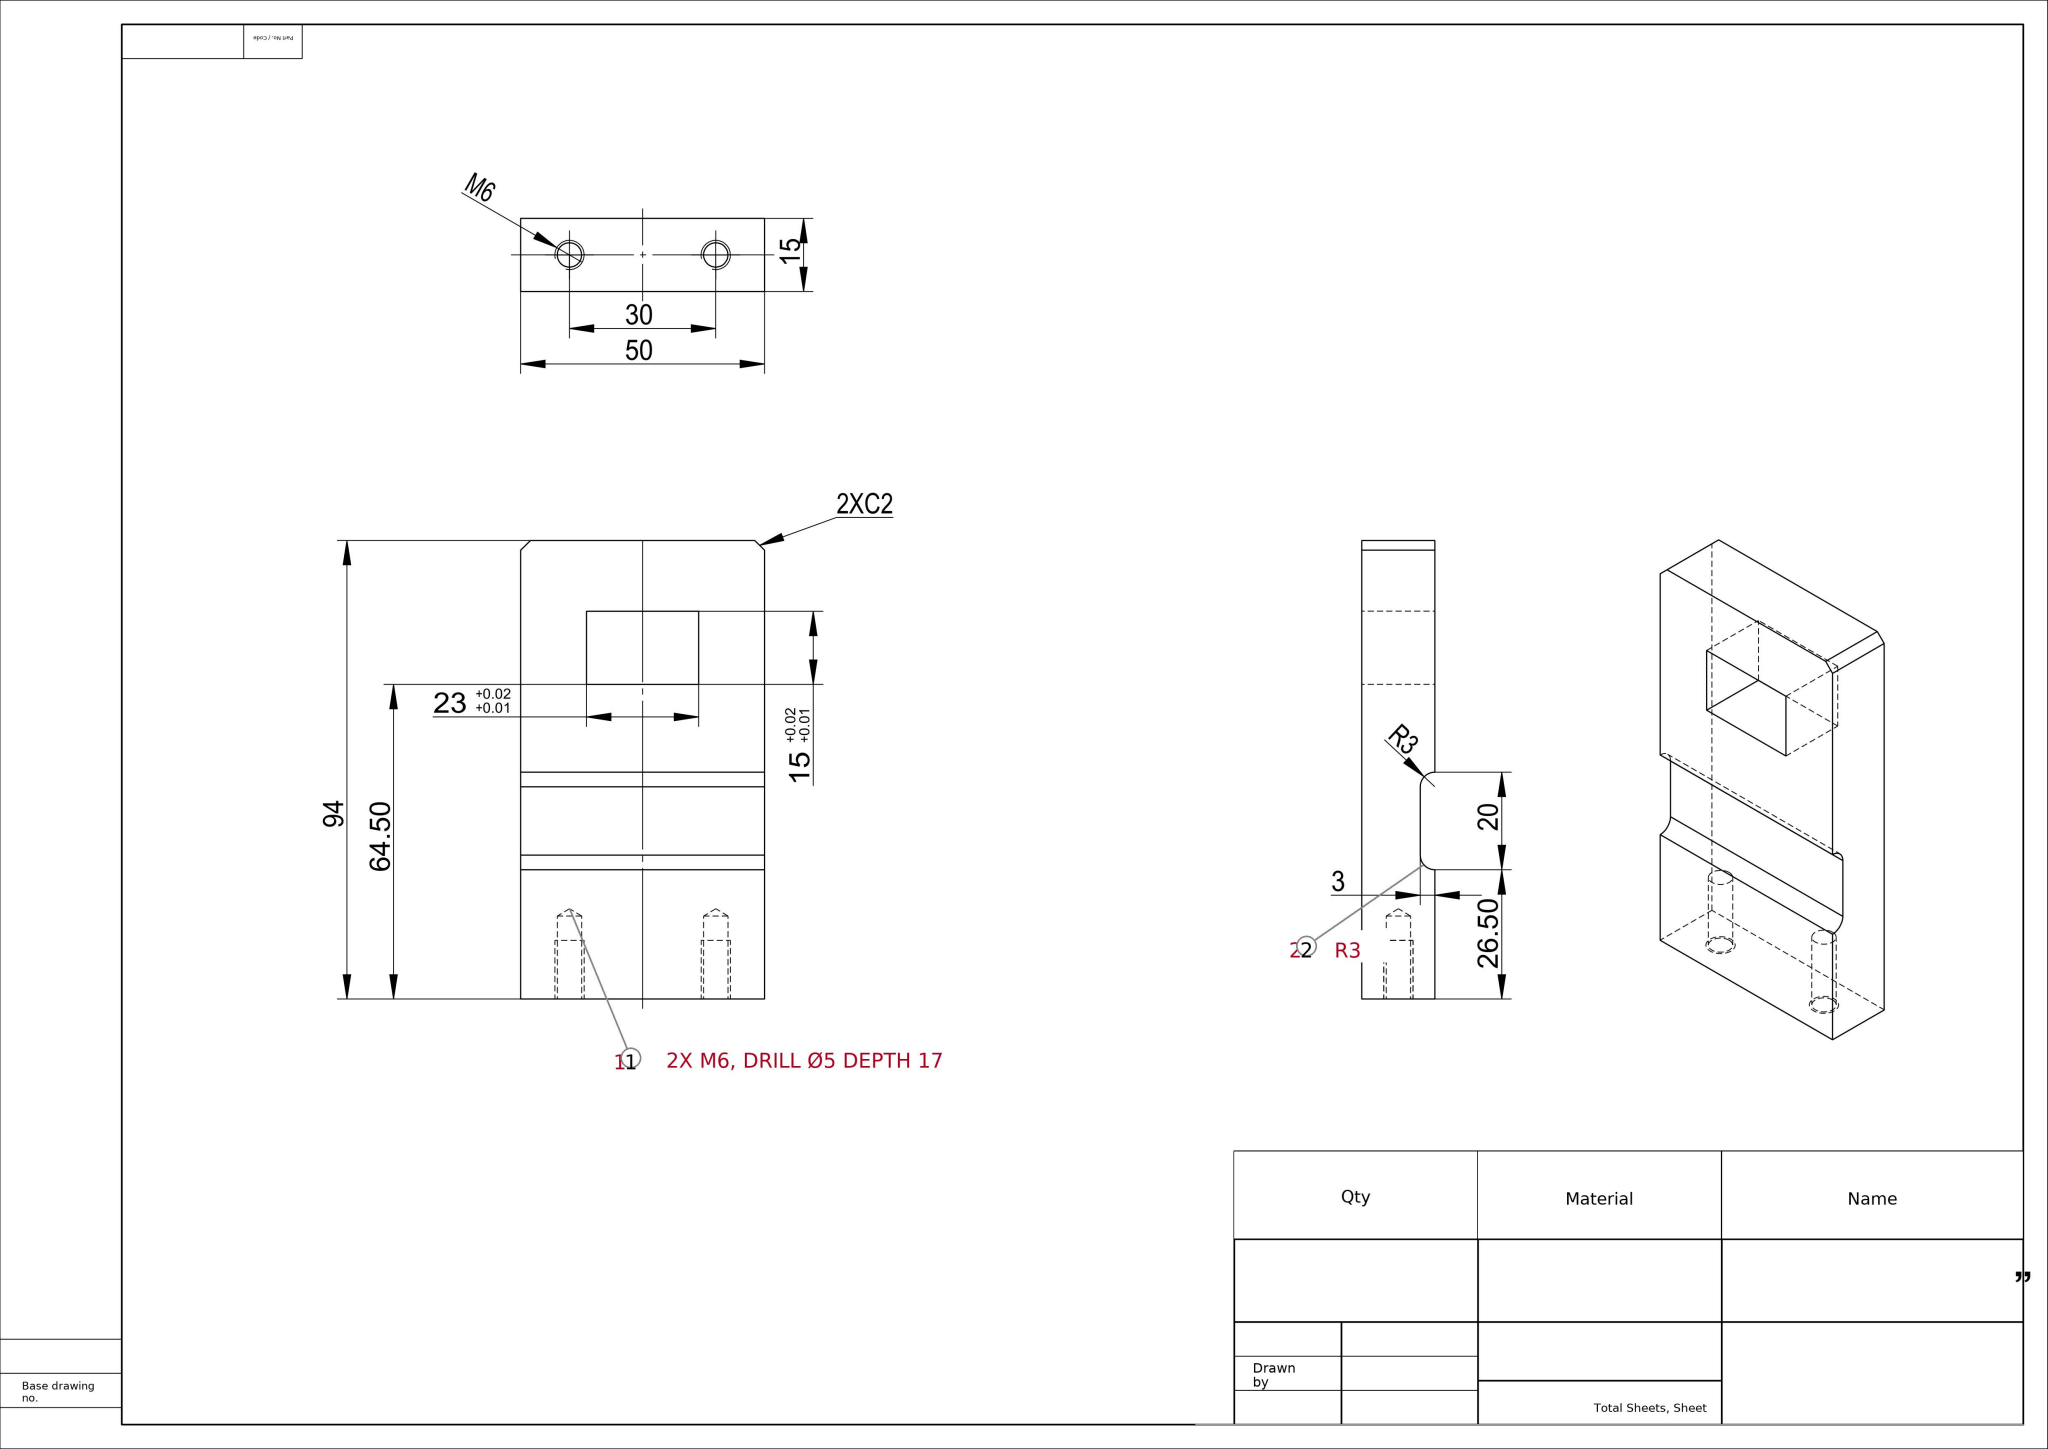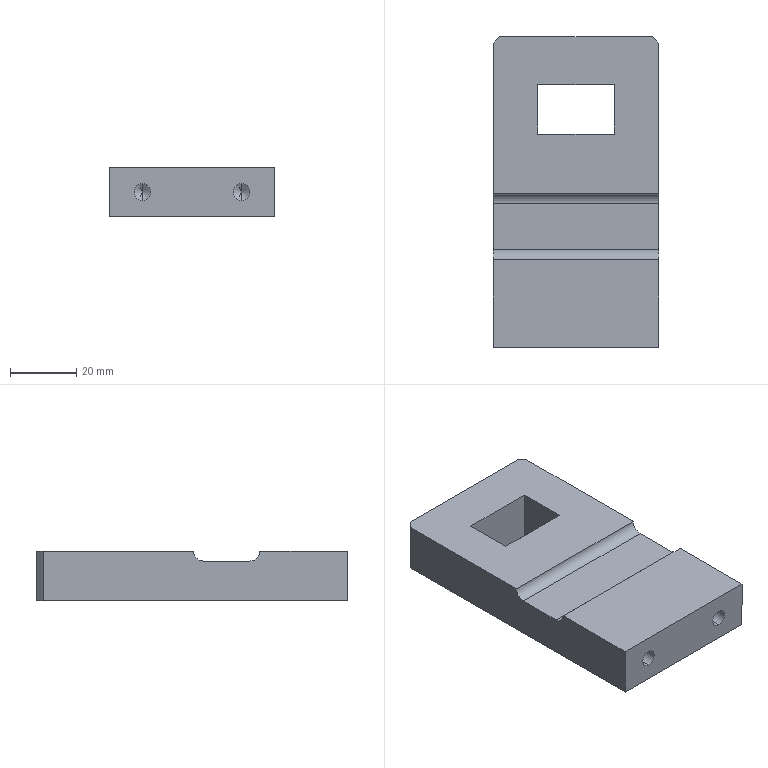Part | SolidWorks | mm | 1 solid | 24 faces | box 50 x 94 x 15 mm | volume 61771 mm3 | plane 14 | cylinder 6 | cone 4 | commonest cylinder face diameters 5 x4 6 x2
STEP:
#1=CARTESIAN_POINT('',(-15.,27.,2.5));
#2=VERTEX_POINT('',#1);
#3=CARTESIAN_POINT('',(-15.,27.,-2.5));
#4=VERTEX_POINT('',#3);
#5=CARTESIAN_POINT('',(-15.,27.,0.));
#6=DIRECTION('',(0.,-1.,0.));
#7=DIRECTION('',(0.,0.,-1.));
#8=AXIS2_PLACEMENT_3D('',#5,#6,#7);
#9=CIRCLE('',#8,2.5);
#10=EDGE_CURVE('',#2,#4,#9,.T.);
#11=ORIENTED_EDGE('',*,*,#10,.F.);
#12=CARTESIAN_POINT('',(-15.,10.,2.5));
#13=VERTEX_POINT('',#12);
#14=CARTESIAN_POINT('',(-15.,10.,2.5));
#15=DIRECTION('',(0.,-1.,0.));
#16=VECTOR('',#15,1000.);
#17=LINE('',#14,#16);
#18=EDGE_CURVE('',#2,#13,#17,.T.);
#19=ORIENTED_EDGE('',*,*,#18,.T.);
#20=CARTESIAN_POINT('',(-15.,10.,-2.5));
#21=VERTEX_POINT('',#20);
#22=CARTESIAN_POINT('',(-15.,10.,0.));
#23=DIRECTION('',(0.,-1.,0.));
#24=DIRECTION('',(0.,0.,-1.));
#25=AXIS2_PLACEMENT_3D('',#22,#23,#24);
#26=CIRCLE('',#25,2.5);
#27=EDGE_CURVE('',#13,#21,#26,.T.);
#28=ORIENTED_EDGE('',*,*,#27,.T.);
#29=CARTESIAN_POINT('',(-15.,10.,-2.5));
#30=DIRECTION('',(0.,-1.,0.));
#31=VECTOR('',#30,1000.);
#32=LINE('',#29,#31);
#33=EDGE_CURVE('',#4,#21,#32,.T.);
#34=ORIENTED_EDGE('',*,*,#33,.F.);
#35=EDGE_LOOP('',(#11,#19,#28,#34));
#36=FACE_OUTER_BOUND('',#35,.T.);
#37=CARTESIAN_POINT('',(-15.,10.,0.));
#38=DIRECTION('',(0.,-1.,0.));
#39=DIRECTION('',(0.,0.,-1.));
#40=AXIS2_PLACEMENT_3D('',#37,#38,#39);
#41=CYLINDRICAL_SURFACE('',#40,2.5);
#42=ADVANCED_FACE('',(#36),#41,.F.);
#43=CARTESIAN_POINT('',(-15.,28.502,0.));
#44=VERTEX_POINT('',#43);
#45=CARTESIAN_POINT('',(-15.,27.,-2.5));
#46=DIRECTION('',(0.,-0.515,-0.8572));
#47=VECTOR('',#46,1000.);
#48=LINE('',#45,#47);
#49=EDGE_CURVE('',#44,#4,#48,.T.);
#50=ORIENTED_EDGE('',*,*,#49,.F.);
#51=CARTESIAN_POINT('',(-15.,27.,2.5));
#52=DIRECTION('',(0.,-0.515,0.8572));
#53=VECTOR('',#52,1000.);
#54=LINE('',#51,#53);
#55=EDGE_CURVE('',#44,#2,#54,.T.);
#56=ORIENTED_EDGE('',*,*,#55,.T.);
#57=ORIENTED_EDGE('',*,*,#10,.T.);
#58=EDGE_LOOP('',(#50,#56,#57));
#59=FACE_OUTER_BOUND('',#58,.T.);
#60=CARTESIAN_POINT('',(-15.,27.,0.));
#61=DIRECTION('',(0.,-1.,0.));
#62=DIRECTION('',(0.,0.,-1.));
#63=AXIS2_PLACEMENT_3D('',#60,#61,#62);
#64=CONICAL_SURFACE('',#63,2.5,1.03);
#65=ADVANCED_FACE('',(#59),#64,.F.);
#66=CARTESIAN_POINT('',(15.,27.,2.5));
#67=VERTEX_POINT('',#66);
#68=CARTESIAN_POINT('',(15.,27.,-2.5));
#69=VERTEX_POINT('',#68);
#70=CARTESIAN_POINT('',(15.,27.,0.));
#71=DIRECTION('',(0.,-1.,0.));
#72=DIRECTION('',(0.,0.,-1.));
#73=AXIS2_PLACEMENT_3D('',#70,#71,#72);
#74=CIRCLE('',#73,2.5);
#75=EDGE_CURVE('',#67,#69,#74,.T.);
#76=ORIENTED_EDGE('',*,*,#75,.F.);
#77=CARTESIAN_POINT('',(15.,10.,2.5));
#78=VERTEX_POINT('',#77);
#79=CARTESIAN_POINT('',(15.,10.,2.5));
#80=DIRECTION('',(0.,-1.,0.));
#81=VECTOR('',#80,1000.);
#82=LINE('',#79,#81);
#83=EDGE_CURVE('',#67,#78,#82,.T.);
#84=ORIENTED_EDGE('',*,*,#83,.T.);
#85=CARTESIAN_POINT('',(15.,10.,-2.5));
#86=VERTEX_POINT('',#85);
#87=CARTESIAN_POINT('',(15.,10.,0.));
#88=DIRECTION('',(0.,-1.,0.));
#89=DIRECTION('',(0.,0.,-1.));
#90=AXIS2_PLACEMENT_3D('',#87,#88,#89);
#91=CIRCLE('',#90,2.5);
#92=EDGE_CURVE('',#78,#86,#91,.T.);
#93=ORIENTED_EDGE('',*,*,#92,.T.);
#94=CARTESIAN_POINT('',(15.,10.,-2.5));
#95=DIRECTION('',(0.,-1.,0.));
#96=VECTOR('',#95,1000.);
#97=LINE('',#94,#96);
#98=EDGE_CURVE('',#69,#86,#97,.T.);
#99=ORIENTED_EDGE('',*,*,#98,.F.);
#100=EDGE_LOOP('',(#76,#84,#93,#99));
#101=FACE_OUTER_BOUND('',#100,.T.);
#102=CARTESIAN_POINT('',(15.,10.,0.));
#103=DIRECTION('',(0.,-1.,0.));
#104=DIRECTION('',(0.,0.,-1.));
#105=AXIS2_PLACEMENT_3D('',#102,#103,#104);
#106=CYLINDRICAL_SURFACE('',#105,2.5);
#107=ADVANCED_FACE('',(#101),#106,.F.);
#108=CARTESIAN_POINT('',(15.,28.502,0.));
#109=VERTEX_POINT('',#108);
#110=CARTESIAN_POINT('',(15.,27.,-2.5));
#111=DIRECTION('',(0.,-0.515,-0.8572));
#112=VECTOR('',#111,1000.);
#113=LINE('',#110,#112);
#114=EDGE_CURVE('',#109,#69,#113,.T.);
#115=ORIENTED_EDGE('',*,*,#114,.F.);
#116=CARTESIAN_POINT('',(15.,27.,2.5));
#117=DIRECTION('',(0.,-0.515,0.8572));
#118=VECTOR('',#117,1000.);
#119=LINE('',#116,#118);
#120=EDGE_CURVE('',#109,#67,#119,.T.);
#121=ORIENTED_EDGE('',*,*,#120,.T.);
#122=ORIENTED_EDGE('',*,*,#75,.T.);
#123=EDGE_LOOP('',(#115,#121,#122));
#124=FACE_OUTER_BOUND('',#123,.T.);
#125=CARTESIAN_POINT('',(15.,27.,0.));
#126=DIRECTION('',(0.,-1.,0.));
#127=DIRECTION('',(0.,0.,-1.));
#128=AXIS2_PLACEMENT_3D('',#125,#126,#127);
#129=CONICAL_SURFACE('',#128,2.5,1.03);
#130=ADVANCED_FACE('',(#124),#129,.F.);
#131=CARTESIAN_POINT('',(25.,102.,-7.5));
#132=VERTEX_POINT('',#131);
#133=CARTESIAN_POINT('',(25.,10.,-7.5));
#134=VERTEX_POINT('',#133);
#135=CARTESIAN_POINT('',(25.,120.,-7.5));
#136=DIRECTION('',(0.,-1.,0.));
#137=VECTOR('',#136,1000.);
#138=LINE('',#135,#137);
#139=EDGE_CURVE('',#132,#134,#138,.T.);
#140=ORIENTED_EDGE('',*,*,#139,.F.);
#141=CARTESIAN_POINT('',(25.,102.,7.5));
#142=VERTEX_POINT('',#141);
#143=CARTESIAN_POINT('',(25.,102.,-7.5));
#144=DIRECTION('',(0.,0.,1.));
#145=VECTOR('',#144,1000.);
#146=LINE('',#143,#145);
#147=EDGE_CURVE('',#132,#142,#146,.T.);
#148=ORIENTED_EDGE('',*,*,#147,.T.);
#149=CARTESIAN_POINT('',(25.,56.5,7.5));
#150=VERTEX_POINT('',#149);
#151=CARTESIAN_POINT('',(25.,120.,7.5));
#152=DIRECTION('',(0.,-1.,0.));
#153=VECTOR('',#152,1000.);
#154=LINE('',#151,#153);
#155=EDGE_CURVE('',#142,#150,#154,.T.);
#156=ORIENTED_EDGE('',*,*,#155,.T.);
#157=CARTESIAN_POINT('',(25.,53.5,4.5));
#158=VERTEX_POINT('',#157);
#159=CARTESIAN_POINT('',(25.,53.5,7.5));
#160=DIRECTION('',(-1.,0.,0.));
#161=DIRECTION('',(0.,0.,1.));
#162=AXIS2_PLACEMENT_3D('',#159,#160,#161);
#163=CIRCLE('',#162,3.);
#164=EDGE_CURVE('',#150,#158,#163,.T.);
#165=ORIENTED_EDGE('',*,*,#164,.T.);
#166=CARTESIAN_POINT('',(25.,39.5,4.5));
#167=VERTEX_POINT('',#166);
#168=CARTESIAN_POINT('',(25.,56.5,4.5));
#169=DIRECTION('',(-0.,-1.,0.));
#170=VECTOR('',#169,1000.);
#171=LINE('',#168,#170);
#172=EDGE_CURVE('',#158,#167,#171,.T.);
#173=ORIENTED_EDGE('',*,*,#172,.T.);
#174=CARTESIAN_POINT('',(25.,36.5,7.5));
#175=VERTEX_POINT('',#174);
#176=CARTESIAN_POINT('',(25.,39.5,7.5));
#177=DIRECTION('',(-1.,0.,0.));
#178=DIRECTION('',(0.,0.,1.));
#179=AXIS2_PLACEMENT_3D('',#176,#177,#178);
#180=CIRCLE('',#179,3.);
#181=EDGE_CURVE('',#167,#175,#180,.T.);
#182=ORIENTED_EDGE('',*,*,#181,.T.);
#183=CARTESIAN_POINT('',(25.,10.,7.5));
#184=VERTEX_POINT('',#183);
#185=CARTESIAN_POINT('',(25.,120.,7.5));
#186=DIRECTION('',(0.,-1.,0.));
#187=VECTOR('',#186,1000.);
#188=LINE('',#185,#187);
#189=EDGE_CURVE('',#175,#184,#188,.T.);
#190=ORIENTED_EDGE('',*,*,#189,.T.);
#191=CARTESIAN_POINT('',(25.,10.,7.5));
#192=DIRECTION('',(0.,0.,-1.));
#193=VECTOR('',#192,1000.);
#194=LINE('',#191,#193);
#195=EDGE_CURVE('',#184,#134,#194,.T.);
#196=ORIENTED_EDGE('',*,*,#195,.T.);
#197=EDGE_LOOP('',(#140,#148,#156,#165,#173,#182,#190,#196));
#198=FACE_OUTER_BOUND('',#197,.T.);
#199=CARTESIAN_POINT('',(25.,120.,-7.5));
#200=DIRECTION('',(-1.,0.,0.));
#201=DIRECTION('',(0.,0.,1.));
#202=AXIS2_PLACEMENT_3D('',#199,#200,#201);
#203=PLANE('',#202);
#204=ADVANCED_FACE('',(#198),#203,.F.);
#205=CARTESIAN_POINT('',(-25.,102.,7.5));
#206=VERTEX_POINT('',#205);
#207=CARTESIAN_POINT('',(-25.,56.5,7.5));
#208=VERTEX_POINT('',#207);
#209=CARTESIAN_POINT('',(-25.,120.,7.5));
#210=DIRECTION('',(0.,-1.,0.));
#211=VECTOR('',#210,1000.);
#212=LINE('',#209,#211);
#213=EDGE_CURVE('',#206,#208,#212,.T.);
#214=ORIENTED_EDGE('',*,*,#213,.F.);
#215=CARTESIAN_POINT('',(-25.,102.,-7.5));
#216=VERTEX_POINT('',#215);
#217=CARTESIAN_POINT('',(-25.,102.,-7.5));
#218=DIRECTION('',(0.,0.,-1.));
#219=VECTOR('',#218,1000.);
#220=LINE('',#217,#219);
#221=EDGE_CURVE('',#206,#216,#220,.T.);
#222=ORIENTED_EDGE('',*,*,#221,.T.);
#223=CARTESIAN_POINT('',(-25.,10.,-7.5));
#224=VERTEX_POINT('',#223);
#225=CARTESIAN_POINT('',(-25.,120.,-7.5));
#226=DIRECTION('',(0.,-1.,0.));
#227=VECTOR('',#226,1000.);
#228=LINE('',#225,#227);
#229=EDGE_CURVE('',#216,#224,#228,.T.);
#230=ORIENTED_EDGE('',*,*,#229,.T.);
#231=CARTESIAN_POINT('',(-25.,10.,7.5));
#232=VERTEX_POINT('',#231);
#233=CARTESIAN_POINT('',(-25.,10.,7.5));
#234=DIRECTION('',(0.,0.,-1.));
#235=VECTOR('',#234,1000.);
#236=LINE('',#233,#235);
#237=EDGE_CURVE('',#232,#224,#236,.T.);
#238=ORIENTED_EDGE('',*,*,#237,.F.);
#239=CARTESIAN_POINT('',(-25.,36.5,7.5));
#240=VERTEX_POINT('',#239);
#241=CARTESIAN_POINT('',(-25.,120.,7.5));
#242=DIRECTION('',(0.,-1.,0.));
#243=VECTOR('',#242,1000.);
#244=LINE('',#241,#243);
#245=EDGE_CURVE('',#240,#232,#244,.T.);
#246=ORIENTED_EDGE('',*,*,#245,.F.);
#247=CARTESIAN_POINT('',(-25.,39.5,4.5));
#248=VERTEX_POINT('',#247);
#249=CARTESIAN_POINT('',(-25.,39.5,7.5));
#250=DIRECTION('',(1.,0.,0.));
#251=DIRECTION('',(0.,0.,-1.));
#252=AXIS2_PLACEMENT_3D('',#249,#250,#251);
#253=CIRCLE('',#252,3.);
#254=EDGE_CURVE('',#240,#248,#253,.T.);
#255=ORIENTED_EDGE('',*,*,#254,.T.);
#256=CARTESIAN_POINT('',(-25.,53.5,4.5));
#257=VERTEX_POINT('',#256);
#258=CARTESIAN_POINT('',(-25.,56.5,4.5));
#259=DIRECTION('',(0.,1.,0.));
#260=VECTOR('',#259,1000.);
#261=LINE('',#258,#260);
#262=EDGE_CURVE('',#248,#257,#261,.T.);
#263=ORIENTED_EDGE('',*,*,#262,.T.);
#264=CARTESIAN_POINT('',(-25.,53.5,7.5));
#265=DIRECTION('',(1.,0.,0.));
#266=DIRECTION('',(0.,0.,-1.));
#267=AXIS2_PLACEMENT_3D('',#264,#265,#266);
#268=CIRCLE('',#267,3.);
#269=EDGE_CURVE('',#257,#208,#268,.T.);
#270=ORIENTED_EDGE('',*,*,#269,.T.);
#271=EDGE_LOOP('',(#214,#222,#230,#238,#246,#255,#263,#270));
#272=FACE_OUTER_BOUND('',#271,.T.);
#273=CARTESIAN_POINT('',(-25.,120.,-7.5));
#274=DIRECTION('',(1.,0.,0.));
#275=DIRECTION('',(0.,0.,-1.));
#276=AXIS2_PLACEMENT_3D('',#273,#274,#275);
#277=PLANE('',#276);
#278=ADVANCED_FACE('',(#272),#277,.F.);
#279=CARTESIAN_POINT('',(25.,36.5,7.5));
#280=DIRECTION('',(-1.,0.,0.));
#281=VECTOR('',#280,1000.);
#282=LINE('',#279,#281);
#283=EDGE_CURVE('',#175,#240,#282,.T.);
#284=ORIENTED_EDGE('',*,*,#283,.T.);
#285=ORIENTED_EDGE('',*,*,#245,.T.);
#286=CARTESIAN_POINT('',(25.,10.,7.5));
#287=DIRECTION('',(1.,0.,0.));
#288=VECTOR('',#287,1000.);
#289=LINE('',#286,#288);
#290=EDGE_CURVE('',#232,#184,#289,.T.);
#291=ORIENTED_EDGE('',*,*,#290,.T.);
#292=ORIENTED_EDGE('',*,*,#189,.F.);
#293=EDGE_LOOP('',(#284,#285,#291,#292));
#294=FACE_OUTER_BOUND('',#293,.T.);
#295=CARTESIAN_POINT('',(-25.,120.,7.5));
#296=DIRECTION('',(0.,0.,-1.));
#297=DIRECTION('',(-1.,0.,0.));
#298=AXIS2_PLACEMENT_3D('',#295,#296,#297);
#299=PLANE('',#298);
#300=ADVANCED_FACE('',(#294),#299,.F.);
#301=CARTESIAN_POINT('',(-11.5,74.5,7.5));
#302=VERTEX_POINT('',#301);
#303=CARTESIAN_POINT('',(11.5,74.5,7.5));
#304=VERTEX_POINT('',#303);
#305=CARTESIAN_POINT('',(-11.5,74.5,7.5));
#306=DIRECTION('',(1.,0.,0.));
#307=VECTOR('',#306,1000.);
#308=LINE('',#305,#307);
#309=EDGE_CURVE('',#302,#304,#308,.T.);
#310=ORIENTED_EDGE('',*,*,#309,.F.);
#311=CARTESIAN_POINT('',(-11.5,89.5,7.5));
#312=VERTEX_POINT('',#311);
#313=CARTESIAN_POINT('',(-11.5,89.5,7.5));
#314=DIRECTION('',(0.,-1.,0.));
#315=VECTOR('',#314,1000.);
#316=LINE('',#313,#315);
#317=EDGE_CURVE('',#312,#302,#316,.T.);
#318=ORIENTED_EDGE('',*,*,#317,.F.);
#319=CARTESIAN_POINT('',(11.5,89.5,7.5));
#320=VERTEX_POINT('',#319);
#321=CARTESIAN_POINT('',(-11.5,89.5,7.5));
#322=DIRECTION('',(-1.,0.,0.));
#323=VECTOR('',#322,1000.);
#324=LINE('',#321,#323);
#325=EDGE_CURVE('',#320,#312,#324,.T.);
#326=ORIENTED_EDGE('',*,*,#325,.F.);
#327=CARTESIAN_POINT('',(11.5,89.5,7.5));
#328=DIRECTION('',(-0.,1.,0.));
#329=VECTOR('',#328,1000.);
#330=LINE('',#327,#329);
#331=EDGE_CURVE('',#304,#320,#330,.T.);
#332=ORIENTED_EDGE('',*,*,#331,.F.);
#333=EDGE_LOOP('',(#310,#318,#326,#332));
#334=FACE_BOUND('',#333,.T.);
#335=CARTESIAN_POINT('',(-23.,104.,7.5));
#336=VERTEX_POINT('',#335);
#337=CARTESIAN_POINT('',(23.,104.,7.5));
#338=VERTEX_POINT('',#337);
#339=CARTESIAN_POINT('',(-25.,104.,7.5));
#340=DIRECTION('',(1.,0.,0.));
#341=VECTOR('',#340,1000.);
#342=LINE('',#339,#341);
#343=EDGE_CURVE('',#336,#338,#342,.T.);
#344=ORIENTED_EDGE('',*,*,#343,.F.);
#345=CARTESIAN_POINT('',(-23.,104.,7.5));
#346=DIRECTION('',(-0.7071,-0.7071,0.));
#347=VECTOR('',#346,1000.);
#348=LINE('',#345,#347);
#349=EDGE_CURVE('',#336,#206,#348,.T.);
#350=ORIENTED_EDGE('',*,*,#349,.T.);
#351=ORIENTED_EDGE('',*,*,#213,.T.);
#352=CARTESIAN_POINT('',(25.,56.5,7.5));
#353=DIRECTION('',(1.,0.,0.));
#354=VECTOR('',#353,1000.);
#355=LINE('',#352,#354);
#356=EDGE_CURVE('',#208,#150,#355,.T.);
#357=ORIENTED_EDGE('',*,*,#356,.T.);
#358=ORIENTED_EDGE('',*,*,#155,.F.);
#359=CARTESIAN_POINT('',(25.,102.,7.5));
#360=DIRECTION('',(-0.7071,0.7071,0.));
#361=VECTOR('',#360,1000.);
#362=LINE('',#359,#361);
#363=EDGE_CURVE('',#142,#338,#362,.T.);
#364=ORIENTED_EDGE('',*,*,#363,.T.);
#365=EDGE_LOOP('',(#344,#350,#351,#357,#358,#364));
#366=FACE_OUTER_BOUND('',#365,.T.);
#367=CARTESIAN_POINT('',(-25.,120.,7.5));
#368=DIRECTION('',(0.,0.,-1.));
#369=DIRECTION('',(-1.,0.,0.));
#370=AXIS2_PLACEMENT_3D('',#367,#368,#369);
#371=PLANE('',#370);
#372=ADVANCED_FACE('',(#334,#366),#371,.F.);
#373=CARTESIAN_POINT('',(11.5,89.5,-7.5));
#374=VERTEX_POINT('',#373);
#375=CARTESIAN_POINT('',(-11.5,89.5,-7.5));
#376=VERTEX_POINT('',#375);
#377=CARTESIAN_POINT('',(-11.5,89.5,-7.5));
#378=DIRECTION('',(-1.,0.,0.));
#379=VECTOR('',#378,1000.);
#380=LINE('',#377,#379);
#381=EDGE_CURVE('',#374,#376,#380,.T.);
#382=ORIENTED_EDGE('',*,*,#381,.T.);
#383=CARTESIAN_POINT('',(-11.5,74.5,-7.5));
#384=VERTEX_POINT('',#383);
#385=CARTESIAN_POINT('',(-11.5,89.5,-7.5));
#386=DIRECTION('',(0.,-1.,0.));
#387=VECTOR('',#386,1000.);
#388=LINE('',#385,#387);
#389=EDGE_CURVE('',#376,#384,#388,.T.);
#390=ORIENTED_EDGE('',*,*,#389,.T.);
#391=CARTESIAN_POINT('',(11.5,74.5,-7.5));
#392=VERTEX_POINT('',#391);
#393=CARTESIAN_POINT('',(-11.5,74.5,-7.5));
#394=DIRECTION('',(1.,0.,0.));
#395=VECTOR('',#394,1000.);
#396=LINE('',#393,#395);
#397=EDGE_CURVE('',#384,#392,#396,.T.);
#398=ORIENTED_EDGE('',*,*,#397,.T.);
#399=CARTESIAN_POINT('',(11.5,89.5,-7.5));
#400=DIRECTION('',(-0.,1.,0.));
#401=VECTOR('',#400,1000.);
#402=LINE('',#399,#401);
#403=EDGE_CURVE('',#392,#374,#402,.T.);
#404=ORIENTED_EDGE('',*,*,#403,.T.);
#405=EDGE_LOOP('',(#382,#390,#398,#404));
#406=FACE_BOUND('',#405,.T.);
#407=ORIENTED_EDGE('',*,*,#229,.F.);
#408=CARTESIAN_POINT('',(-23.,104.,-7.5));
#409=VERTEX_POINT('',#408);
#410=CARTESIAN_POINT('',(-23.,104.,-7.5));
#411=DIRECTION('',(0.7071,0.7071,0.));
#412=VECTOR('',#411,1000.);
#413=LINE('',#410,#412);
#414=EDGE_CURVE('',#216,#409,#413,.T.);
#415=ORIENTED_EDGE('',*,*,#414,.T.);
#416=CARTESIAN_POINT('',(23.,104.,-7.5));
#417=VERTEX_POINT('',#416);
#418=CARTESIAN_POINT('',(-25.,104.,-7.5));
#419=DIRECTION('',(1.,0.,0.));
#420=VECTOR('',#419,1000.);
#421=LINE('',#418,#420);
#422=EDGE_CURVE('',#409,#417,#421,.T.);
#423=ORIENTED_EDGE('',*,*,#422,.T.);
#424=CARTESIAN_POINT('',(25.,102.,-7.5));
#425=DIRECTION('',(0.7071,-0.7071,0.));
#426=VECTOR('',#425,1000.);
#427=LINE('',#424,#426);
#428=EDGE_CURVE('',#417,#132,#427,.T.);
#429=ORIENTED_EDGE('',*,*,#428,.T.);
#430=ORIENTED_EDGE('',*,*,#139,.T.);
#431=CARTESIAN_POINT('',(25.,10.,-7.5));
#432=DIRECTION('',(1.,0.,0.));
#433=VECTOR('',#432,1000.);
#434=LINE('',#431,#433);
#435=EDGE_CURVE('',#224,#134,#434,.T.);
#436=ORIENTED_EDGE('',*,*,#435,.F.);
#437=EDGE_LOOP('',(#407,#415,#423,#429,#430,#436));
#438=FACE_OUTER_BOUND('',#437,.T.);
#439=CARTESIAN_POINT('',(-25.,120.,-7.5));
#440=DIRECTION('',(0.,0.,1.));
#441=DIRECTION('',(1.,0.,0.));
#442=AXIS2_PLACEMENT_3D('',#439,#440,#441);
#443=PLANE('',#442);
#444=ADVANCED_FACE('',(#406,#438),#443,.F.);
#445=ORIENTED_EDGE('',*,*,#317,.T.);
#446=CARTESIAN_POINT('',(-11.5,74.5,-7.5));
#447=DIRECTION('',(0.,0.,1.));
#448=VECTOR('',#447,1000.);
#449=LINE('',#446,#448);
#450=EDGE_CURVE('',#384,#302,#449,.T.);
#451=ORIENTED_EDGE('',*,*,#450,.F.);
#452=ORIENTED_EDGE('',*,*,#389,.F.);
#453=CARTESIAN_POINT('',(-11.5,89.5,-7.5));
#454=DIRECTION('',(0.,0.,1.));
#455=VECTOR('',#454,1000.);
#456=LINE('',#453,#455);
#457=EDGE_CURVE('',#376,#312,#456,.T.);
#458=ORIENTED_EDGE('',*,*,#457,.T.);
#459=EDGE_LOOP('',(#445,#451,#452,#458));
#460=FACE_OUTER_BOUND('',#459,.T.);
#461=CARTESIAN_POINT('',(-11.5,89.5,-7.5));
#462=DIRECTION('',(-1.,-0.,0.));
#463=DIRECTION('',(0.,-1.,0.));
#464=AXIS2_PLACEMENT_3D('',#461,#462,#463);
#465=PLANE('',#464);
#466=ADVANCED_FACE('',(#460),#465,.F.);
#467=ORIENTED_EDGE('',*,*,#325,.T.);
#468=ORIENTED_EDGE('',*,*,#457,.F.);
#469=ORIENTED_EDGE('',*,*,#381,.F.);
#470=CARTESIAN_POINT('',(11.5,89.5,-7.5));
#471=DIRECTION('',(0.,0.,1.));
#472=VECTOR('',#471,1000.);
#473=LINE('',#470,#472);
#474=EDGE_CURVE('',#374,#320,#473,.T.);
#475=ORIENTED_EDGE('',*,*,#474,.T.);
#476=EDGE_LOOP('',(#467,#468,#469,#475));
#477=FACE_OUTER_BOUND('',#476,.T.);
#478=CARTESIAN_POINT('',(-11.5,89.5,-7.5));
#479=DIRECTION('',(0.,1.,0.));
#480=DIRECTION('',(0.,0.,1.));
#481=AXIS2_PLACEMENT_3D('',#478,#479,#480);
#482=PLANE('',#481);
#483=ADVANCED_FACE('',(#477),#482,.F.);
#484=ORIENTED_EDGE('',*,*,#331,.T.);
#485=ORIENTED_EDGE('',*,*,#474,.F.);
#486=ORIENTED_EDGE('',*,*,#403,.F.);
#487=CARTESIAN_POINT('',(11.5,74.5,-7.5));
#488=DIRECTION('',(0.,0.,1.));
#489=VECTOR('',#488,1000.);
#490=LINE('',#487,#489);
#491=EDGE_CURVE('',#392,#304,#490,.T.);
#492=ORIENTED_EDGE('',*,*,#491,.T.);
#493=EDGE_LOOP('',(#484,#485,#486,#492));
#494=FACE_OUTER_BOUND('',#493,.T.);
#495=CARTESIAN_POINT('',(11.5,89.5,-7.5));
#496=DIRECTION('',(1.,0.,0.));
#497=DIRECTION('',(-0.,1.,0.));
#498=AXIS2_PLACEMENT_3D('',#495,#496,#497);
#499=PLANE('',#498);
#500=ADVANCED_FACE('',(#494),#499,.F.);
#501=ORIENTED_EDGE('',*,*,#309,.T.);
#502=ORIENTED_EDGE('',*,*,#491,.F.);
#503=ORIENTED_EDGE('',*,*,#397,.F.);
#504=ORIENTED_EDGE('',*,*,#450,.T.);
#505=EDGE_LOOP('',(#501,#502,#503,#504));
#506=FACE_OUTER_BOUND('',#505,.T.);
#507=CARTESIAN_POINT('',(-11.5,74.5,-7.5));
#508=DIRECTION('',(0.,-1.,0.));
#509=DIRECTION('',(1.,0.,0.));
#510=AXIS2_PLACEMENT_3D('',#507,#508,#509);
#511=PLANE('',#510);
#512=ADVANCED_FACE('',(#506),#511,.F.);
#513=ORIENTED_EDGE('',*,*,#422,.F.);
#514=CARTESIAN_POINT('',(-23.,104.,-7.5));
#515=DIRECTION('',(0.,0.,1.));
#516=VECTOR('',#515,1000.);
#517=LINE('',#514,#516);
#518=EDGE_CURVE('',#409,#336,#517,.T.);
#519=ORIENTED_EDGE('',*,*,#518,.T.);
#520=ORIENTED_EDGE('',*,*,#343,.T.);
#521=CARTESIAN_POINT('',(23.,104.,-7.5));
#522=DIRECTION('',(-0.,0.,-1.));
#523=VECTOR('',#522,1000.);
#524=LINE('',#521,#523);
#525=EDGE_CURVE('',#338,#417,#524,.T.);
#526=ORIENTED_EDGE('',*,*,#525,.T.);
#527=EDGE_LOOP('',(#513,#519,#520,#526));
#528=FACE_OUTER_BOUND('',#527,.T.);
#529=CARTESIAN_POINT('',(-25.,104.,-7.5));
#530=DIRECTION('',(0.,-1.,0.));
#531=DIRECTION('',(0.,0.,-1.));
#532=AXIS2_PLACEMENT_3D('',#529,#530,#531);
#533=PLANE('',#532);
#534=ADVANCED_FACE('',(#528),#533,.F.);
#535=CARTESIAN_POINT('',(-15.,10.,0.));
#536=DIRECTION('',(0.,-1.,0.));
#537=DIRECTION('',(0.,0.,-1.));
#538=AXIS2_PLACEMENT_3D('',#535,#536,#537);
#539=CIRCLE('',#538,2.5);
#540=EDGE_CURVE('',#21,#13,#539,.T.);
#541=ORIENTED_EDGE('',*,*,#540,.F.);
#542=ORIENTED_EDGE('',*,*,#27,.F.);
#543=EDGE_LOOP('',(#541,#542));
#544=FACE_BOUND('',#543,.T.);
#545=CARTESIAN_POINT('',(15.,10.,0.));
#546=DIRECTION('',(0.,-1.,0.));
#547=DIRECTION('',(0.,0.,-1.));
#548=AXIS2_PLACEMENT_3D('',#545,#546,#547);
#549=CIRCLE('',#548,2.5);
#550=EDGE_CURVE('',#86,#78,#549,.T.);
#551=ORIENTED_EDGE('',*,*,#550,.F.);
#552=ORIENTED_EDGE('',*,*,#92,.F.);
#553=EDGE_LOOP('',(#551,#552));
#554=FACE_BOUND('',#553,.T.);
#555=ORIENTED_EDGE('',*,*,#435,.T.);
#556=ORIENTED_EDGE('',*,*,#195,.F.);
#557=ORIENTED_EDGE('',*,*,#290,.F.);
#558=ORIENTED_EDGE('',*,*,#237,.T.);
#559=EDGE_LOOP('',(#555,#556,#557,#558));
#560=FACE_OUTER_BOUND('',#559,.T.);
#561=CARTESIAN_POINT('',(25.,10.,7.5));
#562=DIRECTION('',(-0.,1.,0.));
#563=DIRECTION('',(-1.,-0.,0.));
#564=AXIS2_PLACEMENT_3D('',#561,#562,#563);
#565=PLANE('',#564);
#566=ADVANCED_FACE('',(#544,#554,#560),#565,.F.);
#567=ORIENTED_EDGE('',*,*,#120,.F.);
#568=ORIENTED_EDGE('',*,*,#114,.T.);
#569=CARTESIAN_POINT('',(15.,27.,0.));
#570=DIRECTION('',(0.,-1.,0.));
#571=DIRECTION('',(0.,0.,-1.));
#572=AXIS2_PLACEMENT_3D('',#569,#570,#571);
#573=CIRCLE('',#572,2.5);
#574=EDGE_CURVE('',#69,#67,#573,.T.);
#575=ORIENTED_EDGE('',*,*,#574,.T.);
#576=EDGE_LOOP('',(#567,#568,#575));
#577=FACE_OUTER_BOUND('',#576,.T.);
#578=CARTESIAN_POINT('',(15.,27.,0.));
#579=DIRECTION('',(0.,-1.,0.));
#580=DIRECTION('',(0.,0.,-1.));
#581=AXIS2_PLACEMENT_3D('',#578,#579,#580);
#582=CONICAL_SURFACE('',#581,2.5,1.03);
#583=ADVANCED_FACE('',(#577),#582,.F.);
#584=ORIENTED_EDGE('',*,*,#83,.F.);
#585=ORIENTED_EDGE('',*,*,#574,.F.);
#586=ORIENTED_EDGE('',*,*,#98,.T.);
#587=ORIENTED_EDGE('',*,*,#550,.T.);
#588=EDGE_LOOP('',(#584,#585,#586,#587));
#589=FACE_OUTER_BOUND('',#588,.T.);
#590=CARTESIAN_POINT('',(15.,10.,0.));
#591=DIRECTION('',(0.,-1.,0.));
#592=DIRECTION('',(0.,0.,-1.));
#593=AXIS2_PLACEMENT_3D('',#590,#591,#592);
#594=CYLINDRICAL_SURFACE('',#593,2.5);
#595=ADVANCED_FACE('',(#589),#594,.F.);
#596=ORIENTED_EDGE('',*,*,#55,.F.);
#597=ORIENTED_EDGE('',*,*,#49,.T.);
#598=CARTESIAN_POINT('',(-15.,27.,0.));
#599=DIRECTION('',(0.,-1.,0.));
#600=DIRECTION('',(0.,0.,-1.));
#601=AXIS2_PLACEMENT_3D('',#598,#599,#600);
#602=CIRCLE('',#601,2.5);
#603=EDGE_CURVE('',#4,#2,#602,.T.);
#604=ORIENTED_EDGE('',*,*,#603,.T.);
#605=EDGE_LOOP('',(#596,#597,#604));
#606=FACE_OUTER_BOUND('',#605,.T.);
#607=CARTESIAN_POINT('',(-15.,27.,0.));
#608=DIRECTION('',(0.,-1.,0.));
#609=DIRECTION('',(0.,0.,-1.));
#610=AXIS2_PLACEMENT_3D('',#607,#608,#609);
#611=CONICAL_SURFACE('',#610,2.5,1.03);
#612=ADVANCED_FACE('',(#606),#611,.F.);
#613=ORIENTED_EDGE('',*,*,#18,.F.);
#614=ORIENTED_EDGE('',*,*,#603,.F.);
#615=ORIENTED_EDGE('',*,*,#33,.T.);
#616=ORIENTED_EDGE('',*,*,#540,.T.);
#617=EDGE_LOOP('',(#613,#614,#615,#616));
#618=FACE_OUTER_BOUND('',#617,.T.);
#619=CARTESIAN_POINT('',(-15.,10.,0.));
#620=DIRECTION('',(0.,-1.,0.));
#621=DIRECTION('',(0.,0.,-1.));
#622=AXIS2_PLACEMENT_3D('',#619,#620,#621);
#623=CYLINDRICAL_SURFACE('',#622,2.5);
#624=ADVANCED_FACE('',(#618),#623,.F.);
#625=ORIENTED_EDGE('',*,*,#262,.F.);
#626=CARTESIAN_POINT('',(0.,39.5,4.5));
#627=DIRECTION('',(1.,0.,0.));
#628=VECTOR('',#627,1000.);
#629=LINE('',#626,#628);
#630=EDGE_CURVE('',#248,#167,#629,.T.);
#631=ORIENTED_EDGE('',*,*,#630,.T.);
#632=ORIENTED_EDGE('',*,*,#172,.F.);
#633=CARTESIAN_POINT('',(0.,53.5,4.5));
#634=DIRECTION('',(-1.,0.,0.));
#635=VECTOR('',#634,1000.);
#636=LINE('',#633,#635);
#637=EDGE_CURVE('',#158,#257,#636,.T.);
#638=ORIENTED_EDGE('',*,*,#637,.T.);
#639=EDGE_LOOP('',(#625,#631,#632,#638));
#640=FACE_OUTER_BOUND('',#639,.T.);
#641=CARTESIAN_POINT('',(0.,0.,4.5));
#642=DIRECTION('',(0.,0.,-1.));
#643=DIRECTION('',(-1.,0.,0.));
#644=AXIS2_PLACEMENT_3D('',#641,#642,#643);
#645=PLANE('',#644);
#646=ADVANCED_FACE('',(#640),#645,.F.);
#647=ORIENTED_EDGE('',*,*,#181,.F.);
#648=ORIENTED_EDGE('',*,*,#630,.F.);
#649=ORIENTED_EDGE('',*,*,#254,.F.);
#650=ORIENTED_EDGE('',*,*,#283,.F.);
#651=EDGE_LOOP('',(#647,#648,#649,#650));
#652=FACE_OUTER_BOUND('',#651,.T.);
#653=CARTESIAN_POINT('',(25.,39.5,7.5));
#654=DIRECTION('',(-1.,0.,0.));
#655=DIRECTION('',(0.,0.,1.));
#656=AXIS2_PLACEMENT_3D('',#653,#654,#655);
#657=CYLINDRICAL_SURFACE('',#656,3.);
#658=ADVANCED_FACE('',(#652),#657,.F.);
#659=ORIENTED_EDGE('',*,*,#269,.F.);
#660=ORIENTED_EDGE('',*,*,#637,.F.);
#661=ORIENTED_EDGE('',*,*,#164,.F.);
#662=ORIENTED_EDGE('',*,*,#356,.F.);
#663=EDGE_LOOP('',(#659,#660,#661,#662));
#664=FACE_OUTER_BOUND('',#663,.T.);
#665=CARTESIAN_POINT('',(25.,53.5,7.5));
#666=DIRECTION('',(1.,0.,0.));
#667=DIRECTION('',(0.,0.,-1.));
#668=AXIS2_PLACEMENT_3D('',#665,#666,#667);
#669=CYLINDRICAL_SURFACE('',#668,3.);
#670=ADVANCED_FACE('',(#664),#669,.F.);
#671=ORIENTED_EDGE('',*,*,#414,.F.);
#672=ORIENTED_EDGE('',*,*,#221,.F.);
#673=ORIENTED_EDGE('',*,*,#349,.F.);
#674=ORIENTED_EDGE('',*,*,#518,.F.);
#675=EDGE_LOOP('',(#671,#672,#673,#674));
#676=FACE_OUTER_BOUND('',#675,.T.);
#677=CARTESIAN_POINT('',(-23.,104.,-7.5));
#678=DIRECTION('',(0.7071,-0.7071,0.));
#679=DIRECTION('',(0.,0.,1.));
#680=AXIS2_PLACEMENT_3D('',#677,#678,#679);
#681=PLANE('',#680);
#682=ADVANCED_FACE('',(#676),#681,.F.);
#683=ORIENTED_EDGE('',*,*,#428,.F.);
#684=ORIENTED_EDGE('',*,*,#525,.F.);
#685=ORIENTED_EDGE('',*,*,#363,.F.);
#686=ORIENTED_EDGE('',*,*,#147,.F.);
#687=EDGE_LOOP('',(#683,#684,#685,#686));
#688=FACE_OUTER_BOUND('',#687,.T.);
#689=CARTESIAN_POINT('',(25.,102.,-7.5));
#690=DIRECTION('',(-0.7071,-0.7071,0.));
#691=DIRECTION('',(0.,0.,1.));
#692=AXIS2_PLACEMENT_3D('',#689,#690,#691);
#693=PLANE('',#692);
#694=ADVANCED_FACE('',(#688),#693,.F.);
#695=CLOSED_SHELL('',(#42,#65,#107,#130,#204,#278,#300,#372,#444,#466,#483,#500,#512,#534,#566,#583,#595,#612,#624,#646,#658,#670,#682,#694));
#696=MANIFOLD_SOLID_BREP('',#695);
#697=CARTESIAN_POINT('',(0.,0.,0.));
#698=DIRECTION('',(0.,0.,1.));
#699=DIRECTION('',(1.,0.,0.));
#700=AXIS2_PLACEMENT_3D('',#697,#698,#699);
#701=(LENGTH_UNIT()NAMED_UNIT(*)SI_UNIT(.MILLI.,.METRE.));
#702=UNCERTAINTY_MEASURE_WITH_UNIT(LENGTH_MEASURE(0.00001),#701,'','');
#703=(NAMED_UNIT(*)PLANE_ANGLE_UNIT()SI_UNIT($,.RADIAN.));
#704=(NAMED_UNIT(*)SI_UNIT($,.STERADIAN.)SOLID_ANGLE_UNIT());
#705=(GEOMETRIC_REPRESENTATION_CONTEXT(3)GLOBAL_UNCERTAINTY_ASSIGNED_CONTEXT((#702))GLOBAL_UNIT_ASSIGNED_CONTEXT((#701,#703,#704))REPRESENTATION_CONTEXT('',''));
#706=ADVANCED_BREP_SHAPE_REPRESENTATION('',(#696,#700),#705);